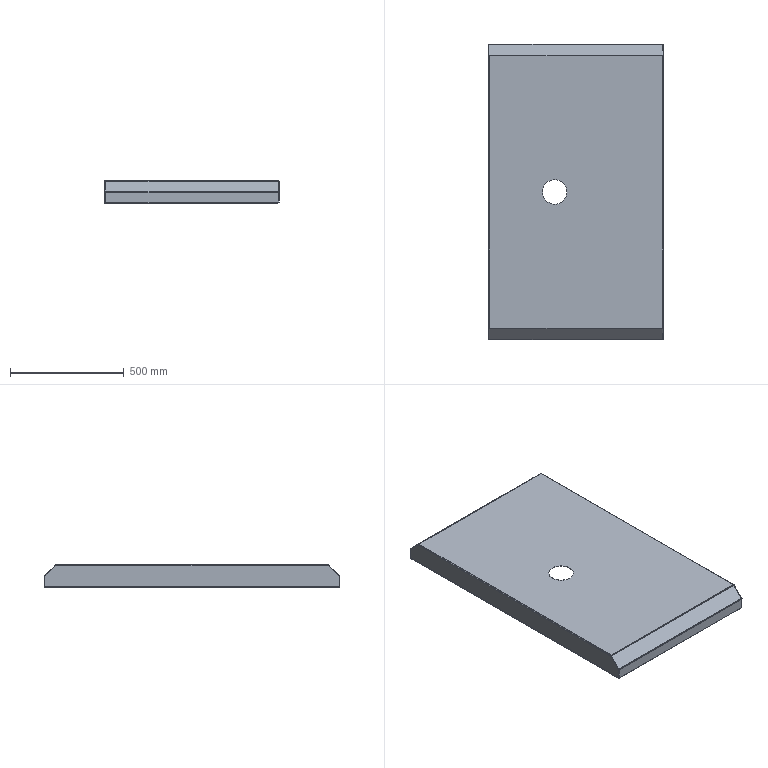Component | SolidWorks | FrontTopCoverAssembly-1_FrontTopCover-1 | 1 solid | 182 faces | volume 2695756 mm3 | plane 120 | cylinder 54 | spline 8 | commonest cylinder face diameters 10 x24 4 x15 8 x13 108 x2 | material Plain Carbon Steel